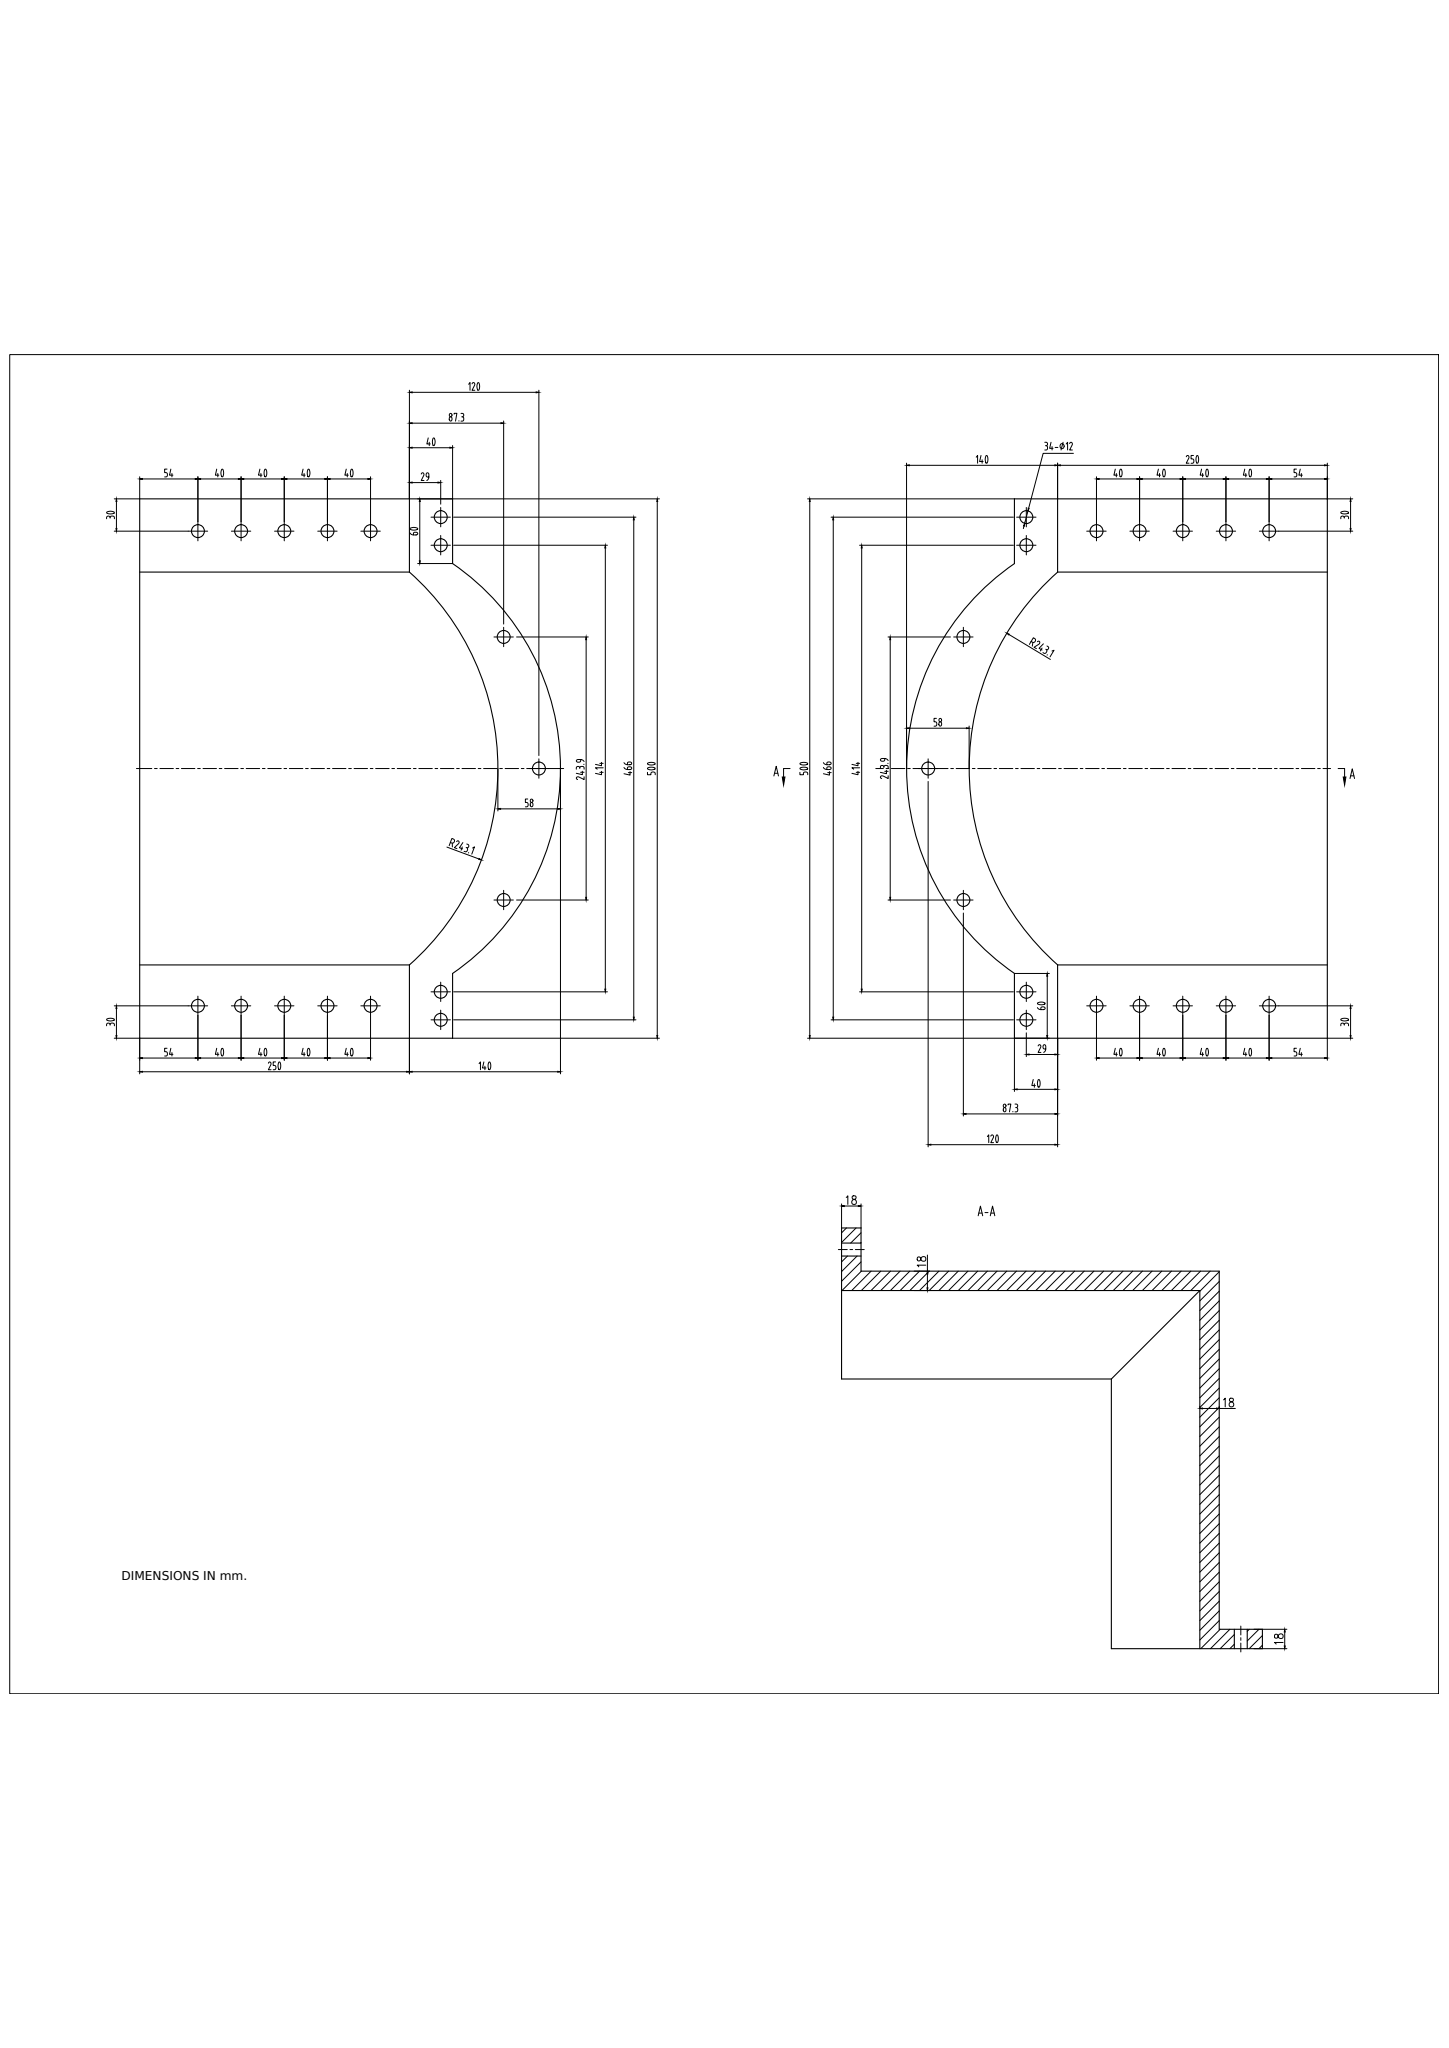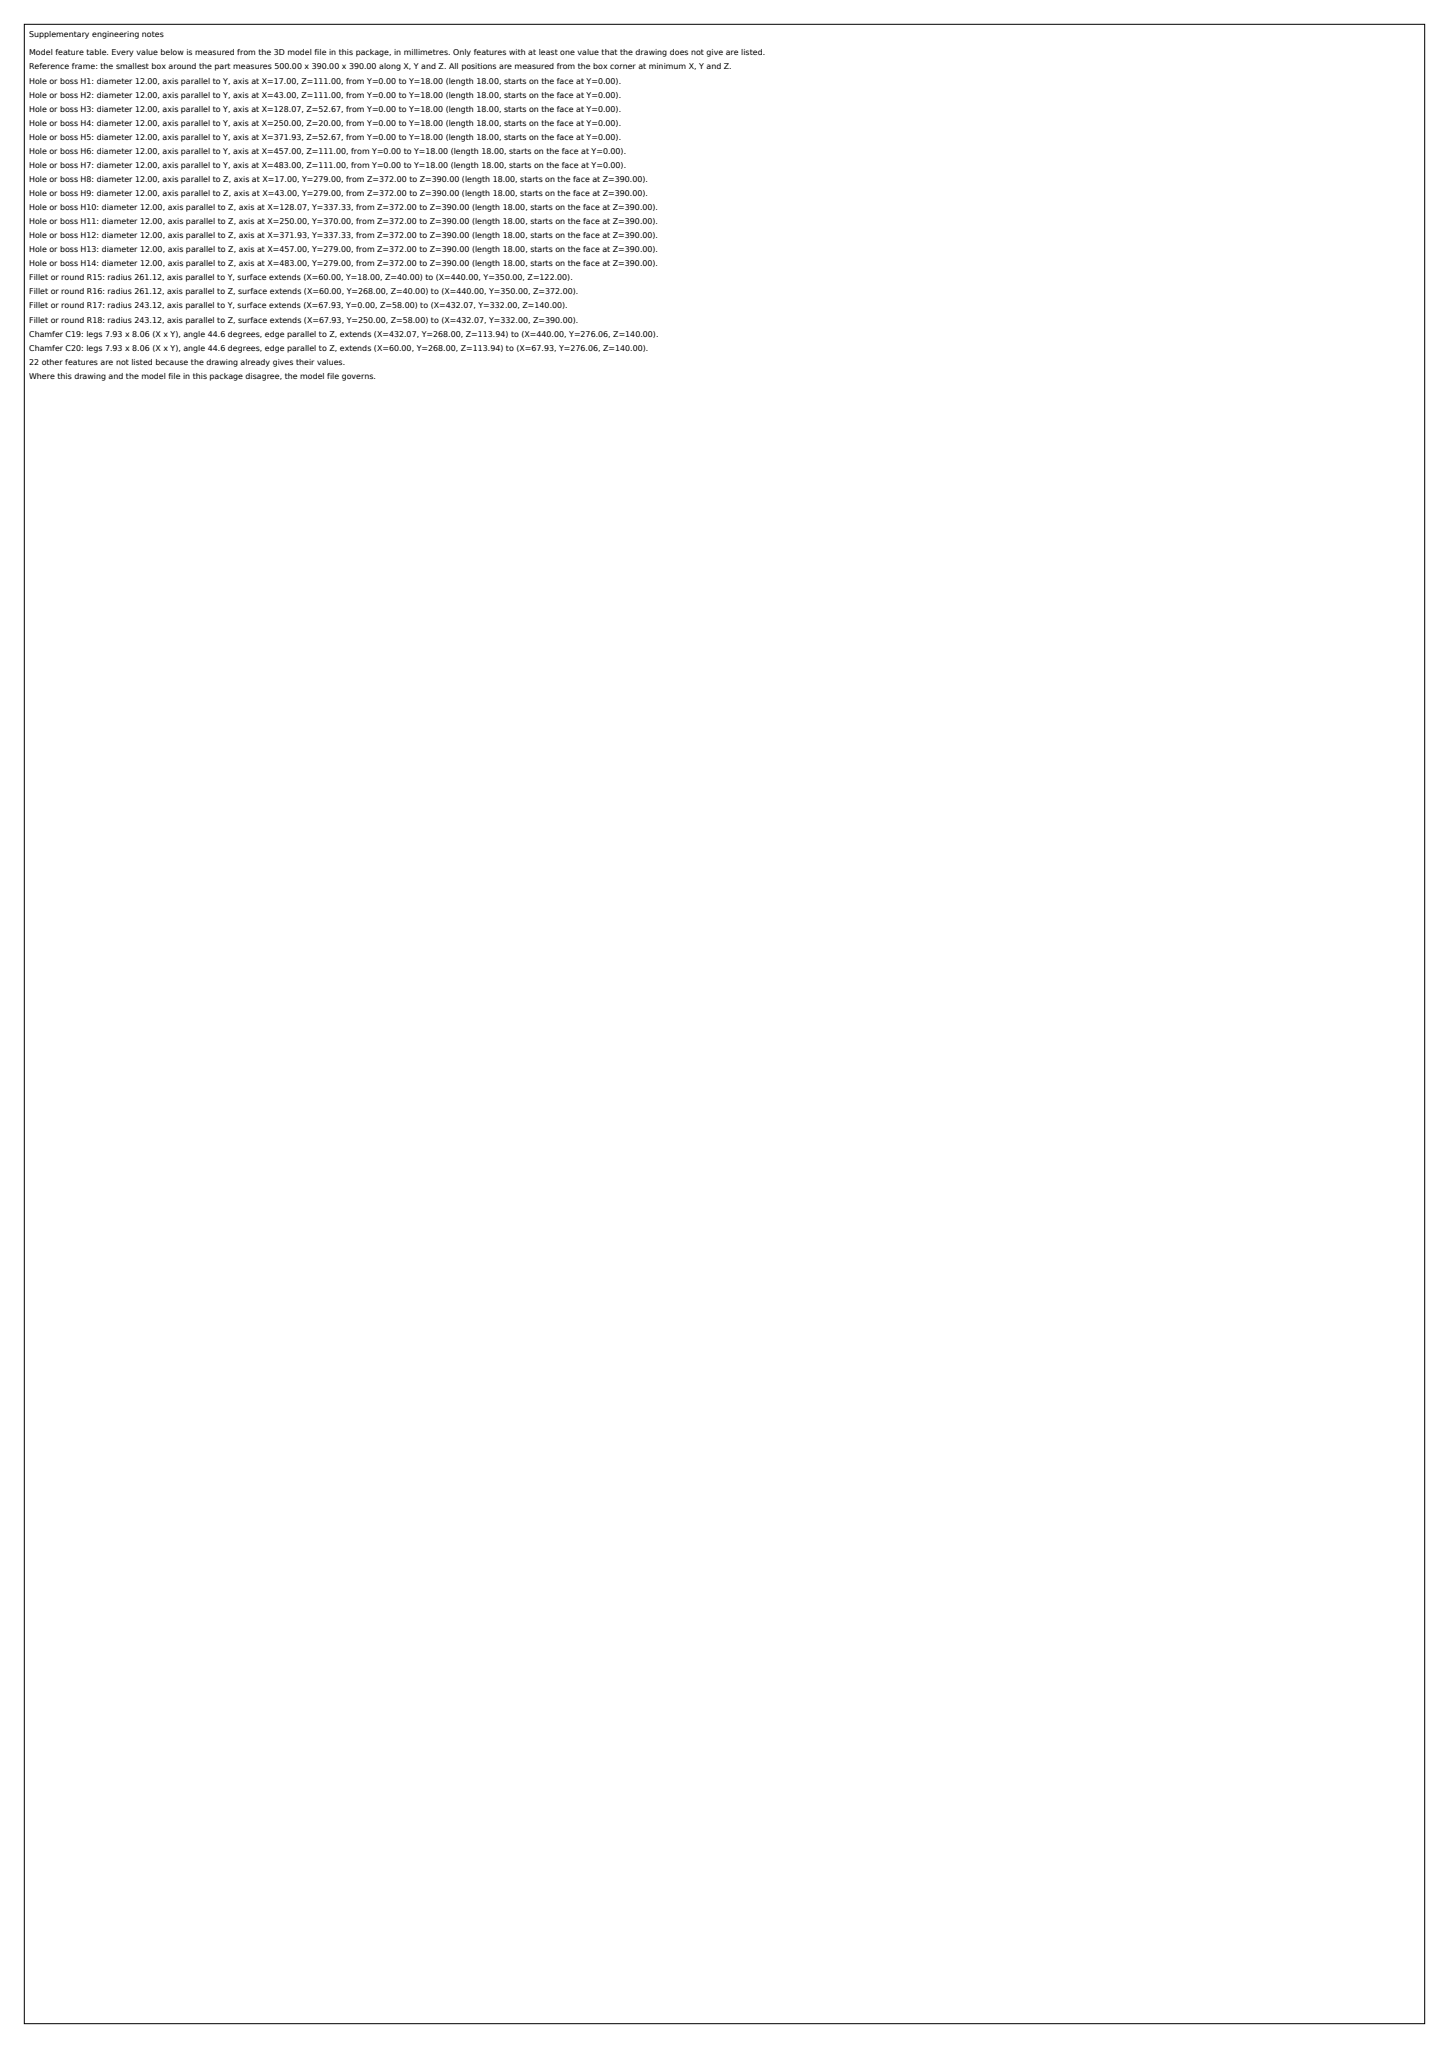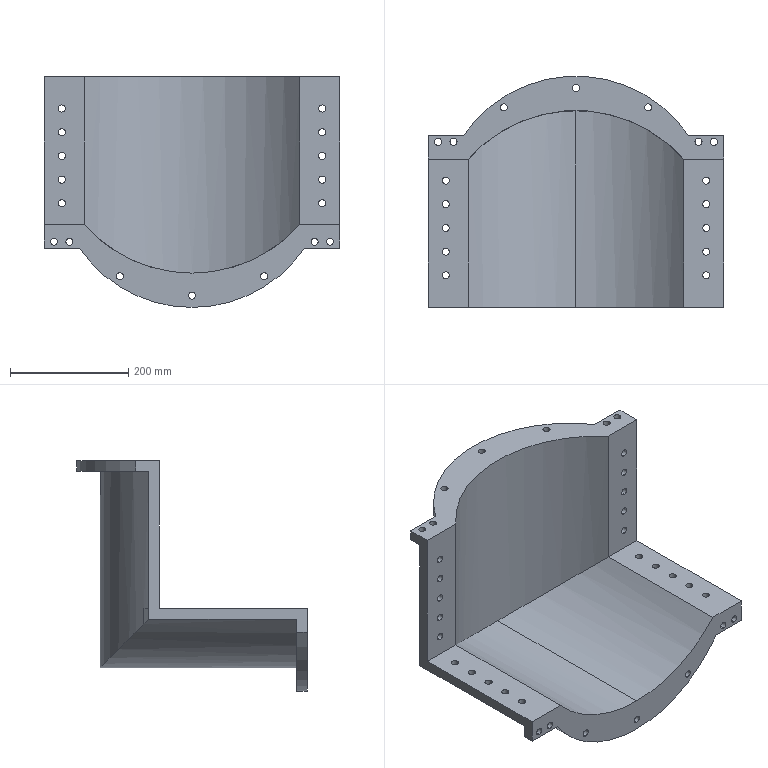Part | SolidWorks | mm | 1 solid | 99 faces | box 500 x 390 x 390 mm | volume 6421614 mm3 | cylinder 77 | plane 22 | commonest cylinder face diameters 12 x68 461 x3 522.244 x3 486.244 x3